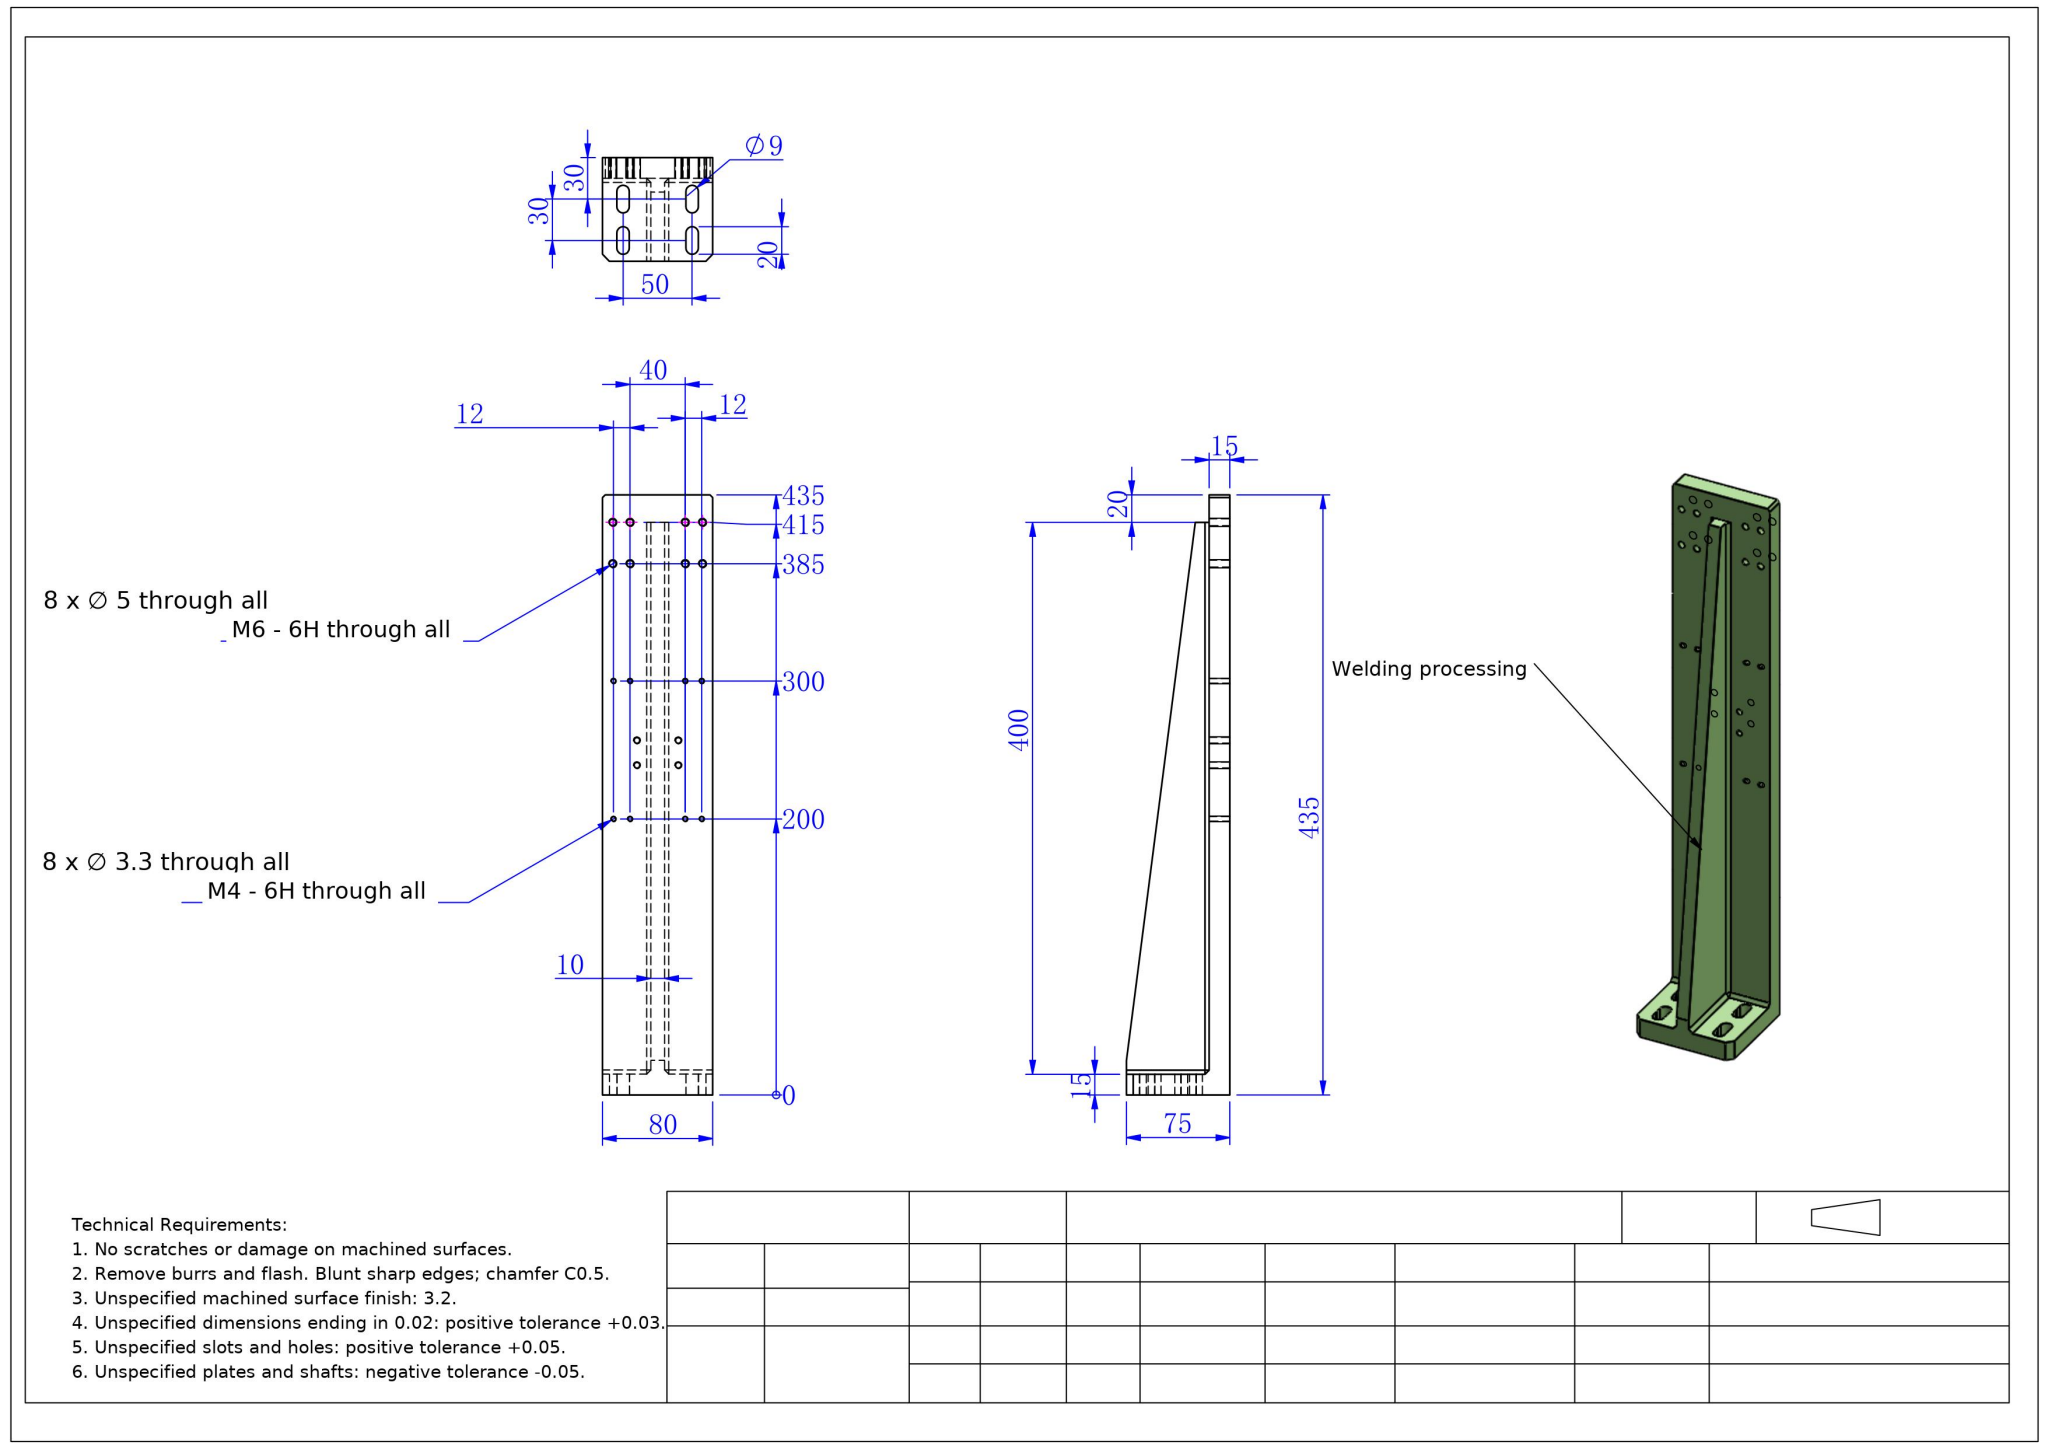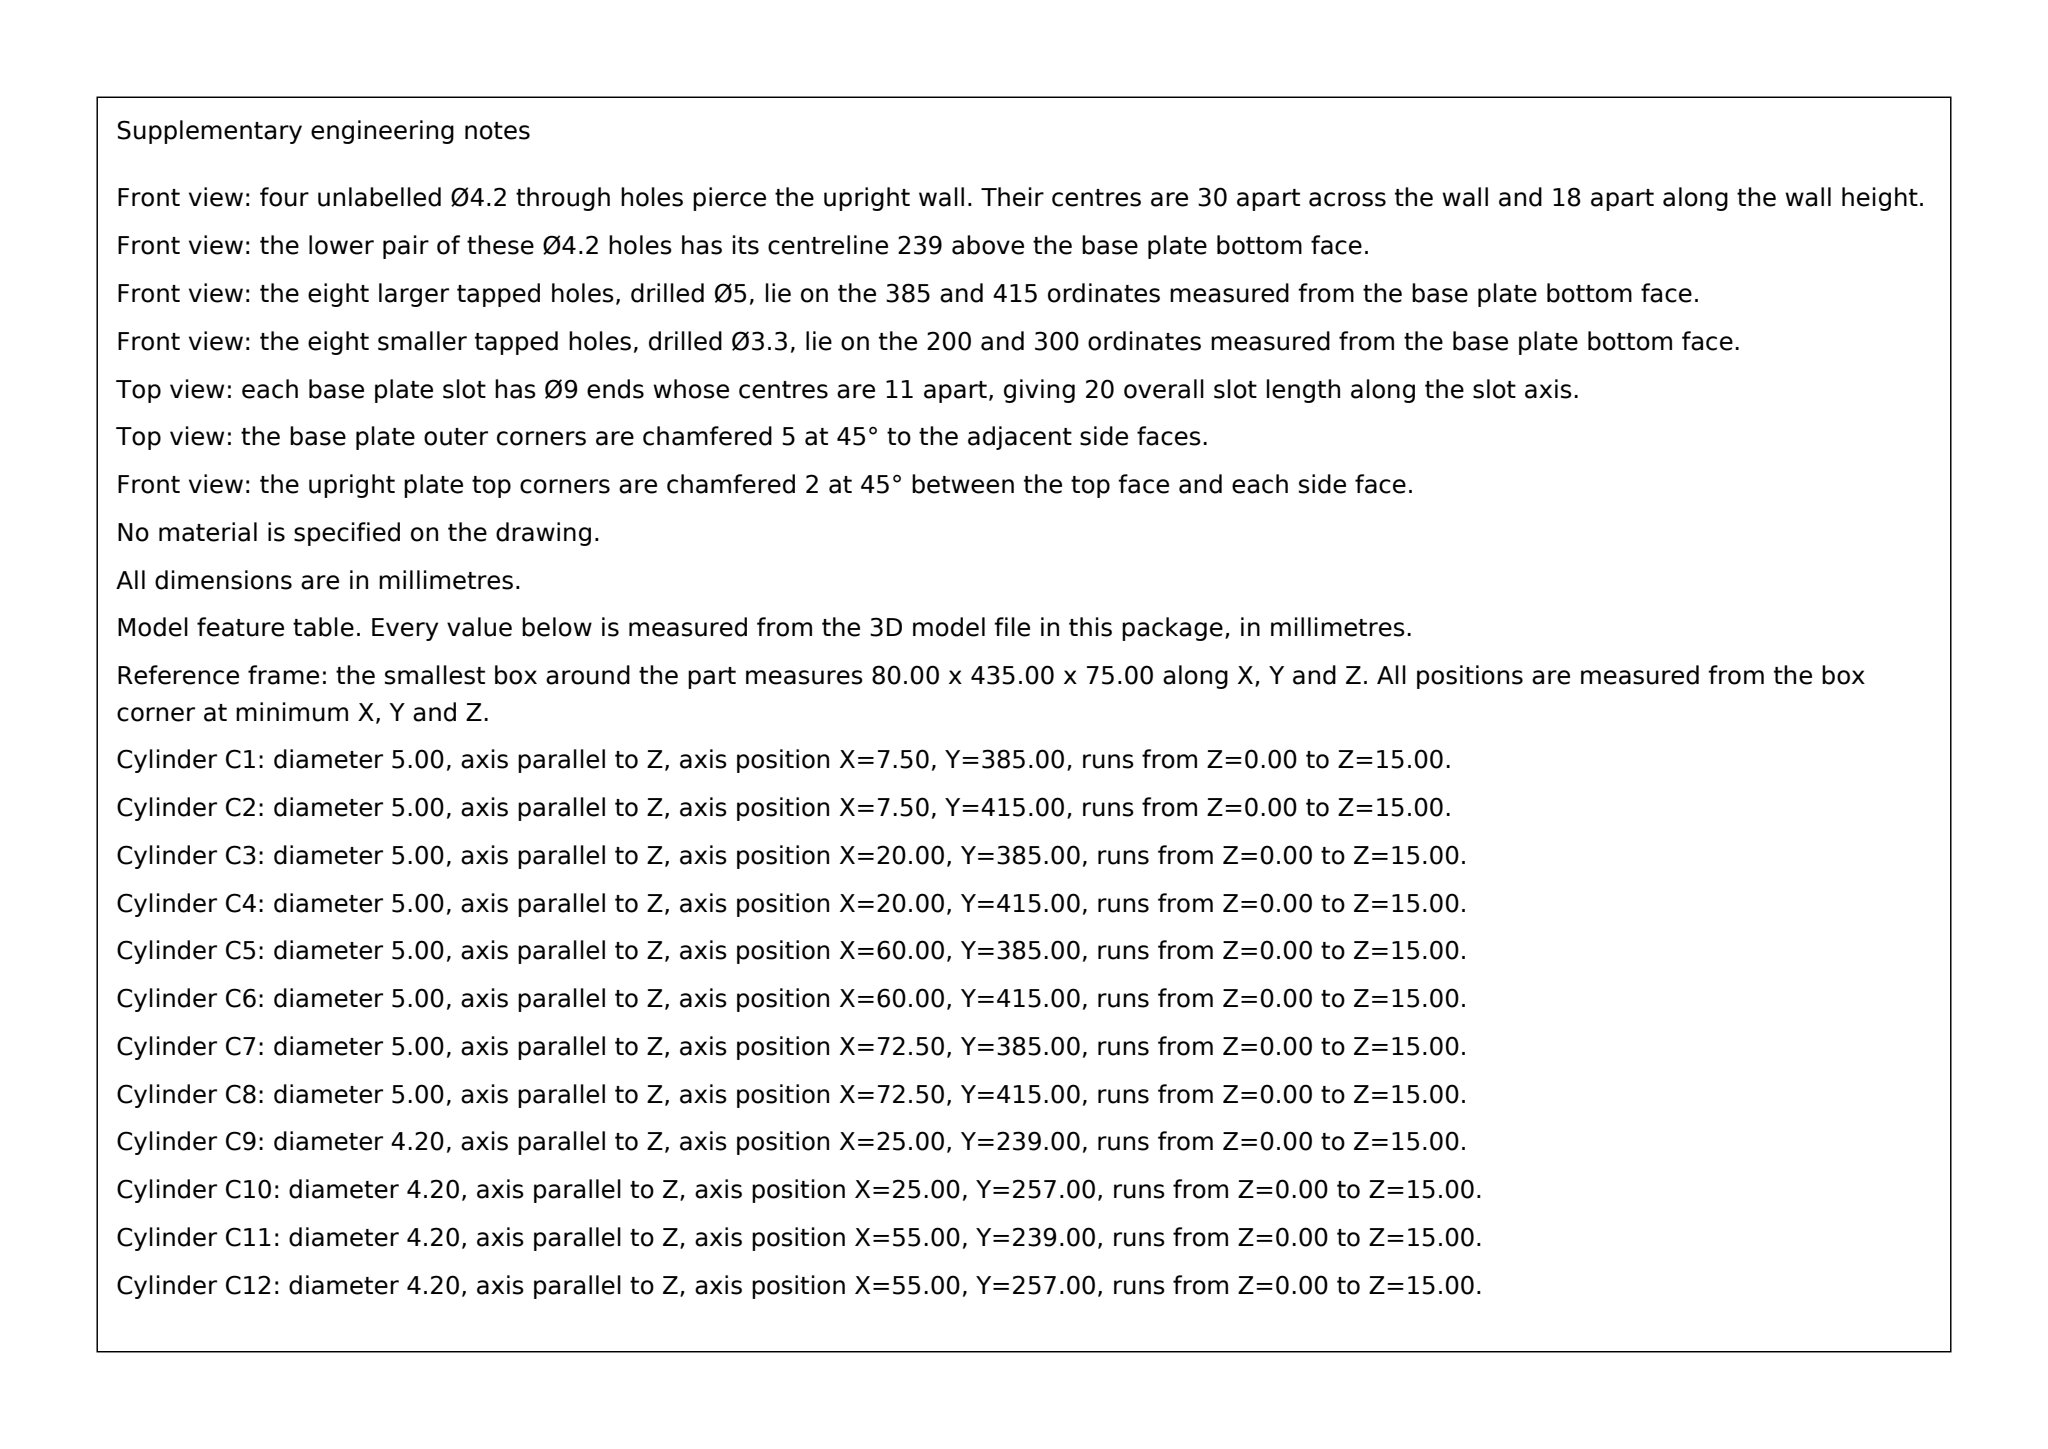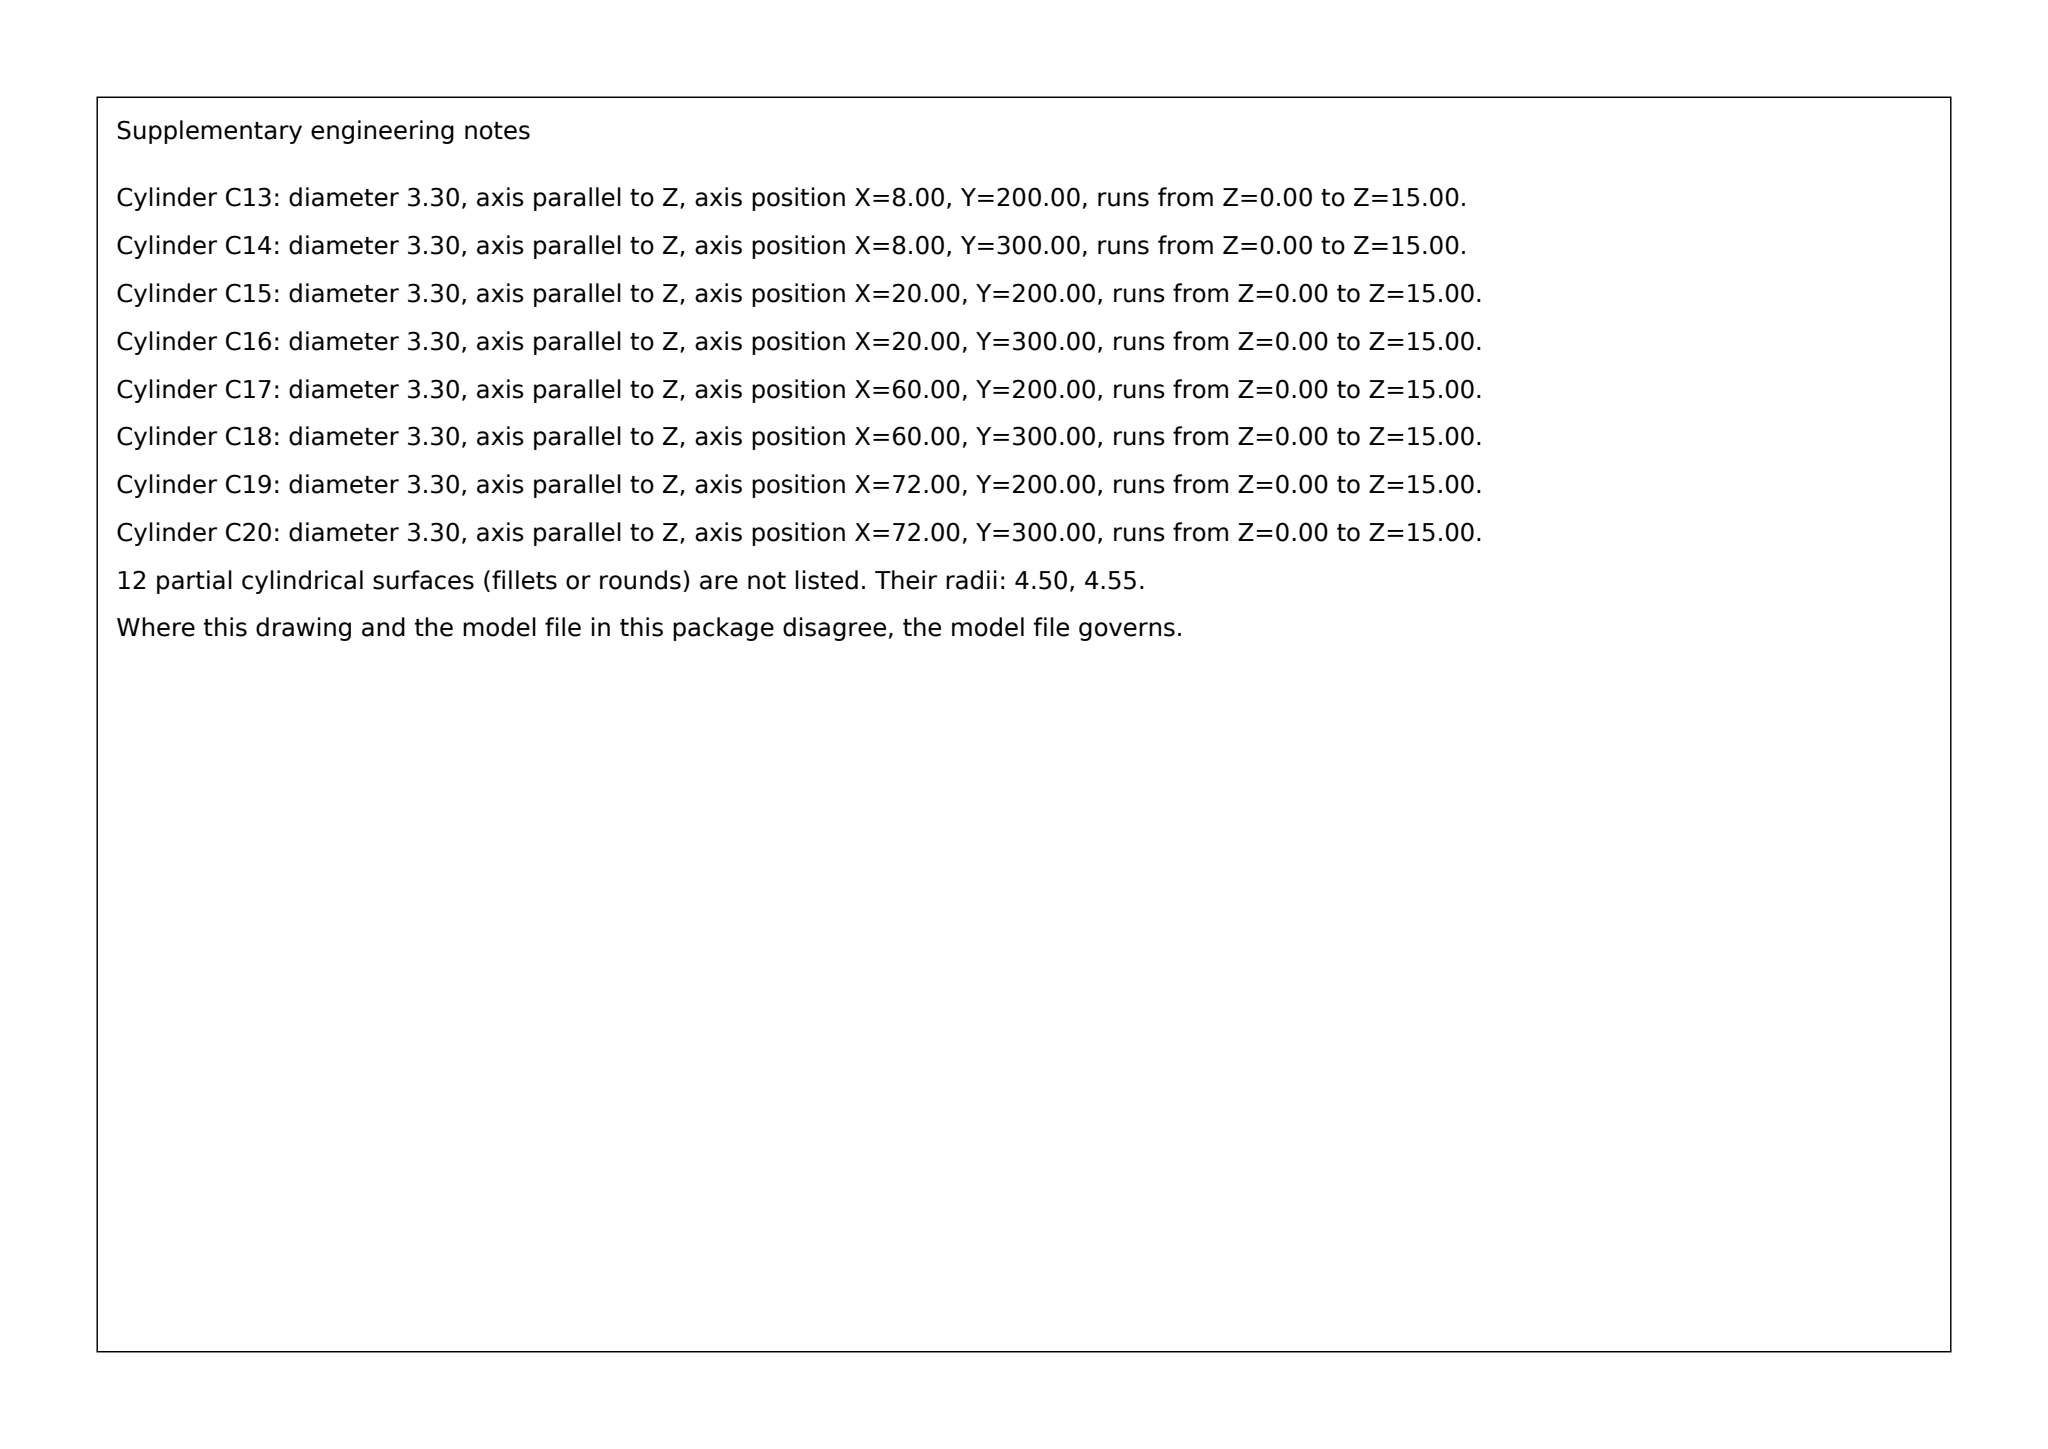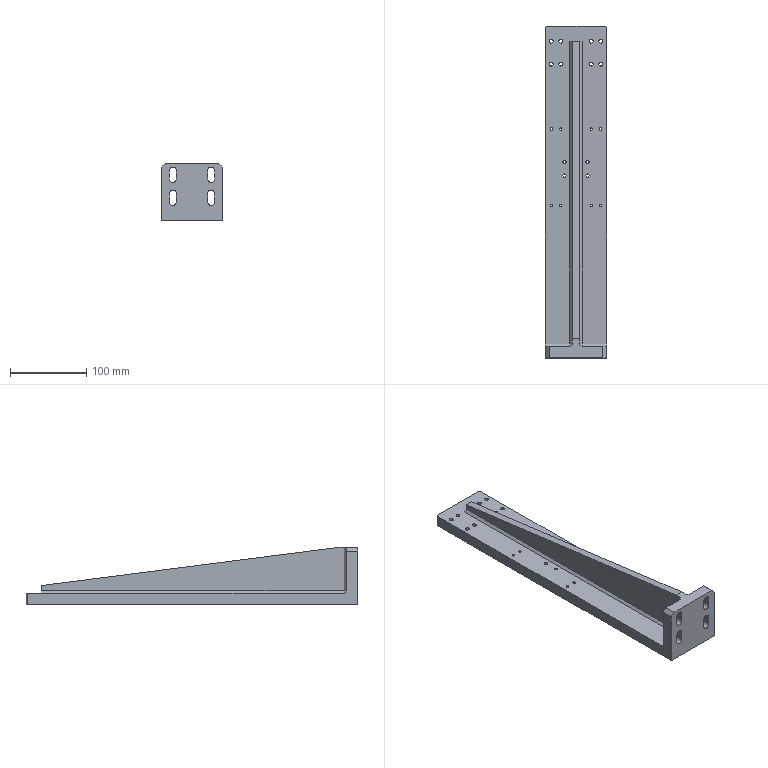Part | SolidWorks | mm | 1 solid | 101 faces | box 80 x 435 x 75 mm | volume 726508 mm3 | cylinder 60 | plane 41 | commonest cylinder face diameters 3.3 x16 5 x16 9 x12 4.2 x8 9.1 x8